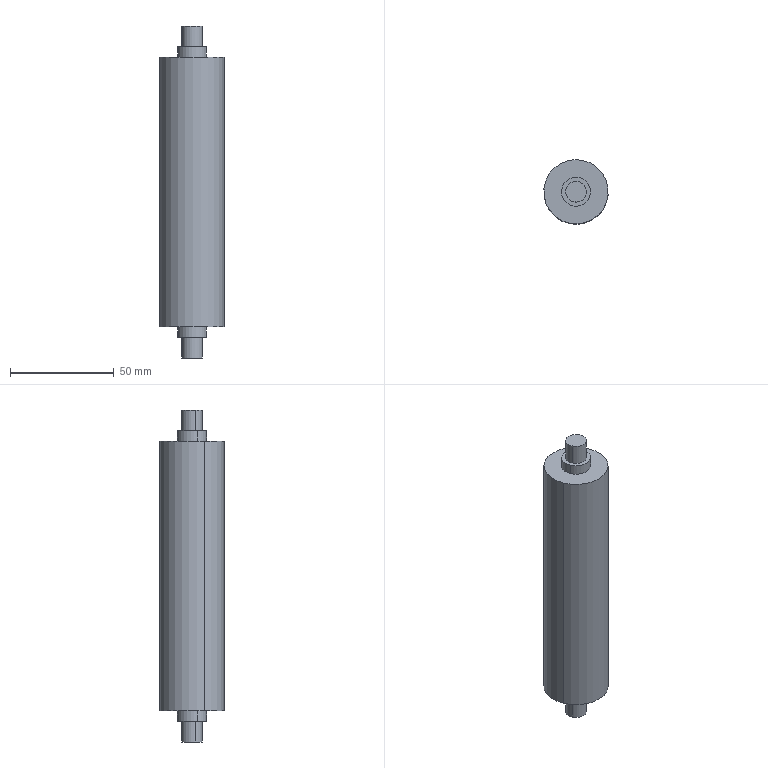Component | SolidWorks | RubberRoller.1-1 | 1 solid | 16 faces | box 31 x 31 x 160 mm | volume 101230 mm3 | cylinder 10 | plane 6 | commonest cylinder face diameters 14 x4 10 x4 31 x2
build123d program:
from build123d import *

# Parameters (mm, degrees)
SKETCH1_2_R         = 16
BOSS_EXTRUDE1_DEPTH = 65
SKETCH2_R           = 7
BOSS_EXTRUDE2_DEPTH = 70
SKETCH4_R           = 5
BOSS_EXTRUDE4_DEPTH = 80
SKETCH1_R           = 17.5
SKETCH1_R_2         = 15.5
CUT_EXTRUDE1_DEPTH  = 70


with BuildPart() as part:
    # Sketch1_2 → Boss-Extrude1 (new, symmetric)
    with BuildSketch(Plane.XY):
        Circle(SKETCH1_2_R)
    extrude(amount=BOSS_EXTRUDE1_DEPTH, both=True)

    # Sketch2 → Boss-Extrude2 (add, symmetric)
    with BuildSketch(Plane.XY):
        Circle(SKETCH2_R)
    extrude(amount=BOSS_EXTRUDE2_DEPTH, both=True)

    # Sketch4 → Boss-Extrude4 (add, symmetric)
    with BuildSketch(Plane.XY):
        Circle(SKETCH4_R)
    extrude(amount=BOSS_EXTRUDE4_DEPTH, both=True)

    # Sketch1 → Cut-Extrude1 (cut, symmetric)
    with BuildSketch(Plane.XY):
        Circle(SKETCH1_R)
        Circle(SKETCH1_R_2, mode=Mode.SUBTRACT)
    extrude(amount=CUT_EXTRUDE1_DEPTH, both=True, mode=Mode.SUBTRACT)


solid = part.part

# Placed as in the assembly
solid = solid.moved(Location((40.5, 166.5, 0), (0, 0, 0)))
STEP:
#1=COLOUR_RGB('',0.7922,0.8196,0.9333);
#2=FILL_AREA_STYLE_COLOUR('',#1);
#3=FILL_AREA_STYLE('',(#2));
#4=SURFACE_STYLE_FILL_AREA(#3);
#5=SURFACE_SIDE_STYLE('',(#4));
#6=SURFACE_STYLE_USAGE(.BOTH.,#5);
#7=PRESENTATION_STYLE_ASSIGNMENT((#6));
#8=CARTESIAN_POINT('',(1.34,6.45,2.559));
#9=VERTEX_POINT('',#8);
#10=CARTESIAN_POINT('',(1.849,6.661,2.559));
#11=VERTEX_POINT('',#10);
#12=CARTESIAN_POINT('',(1.594,6.555,2.559));
#13=DIRECTION('',(0.,0.,1.));
#14=DIRECTION('',(0.9237,0.383,0.));
#15=AXIS2_PLACEMENT_3D('',#12,#13,#14);
#16=CIRCLE('',#15,0.2756);
#17=EDGE_CURVE('',#9,#11,#16,.T.);
#18=ORIENTED_EDGE('',*,*,#17,.T.);
#19=CARTESIAN_POINT('',(1.849,6.661,2.756));
#20=VERTEX_POINT('',#19);
#21=CARTESIAN_POINT('',(1.849,6.661,-2.756));
#22=DIRECTION('',(0.,0.,1.));
#23=VECTOR('',#22,39.37);
#24=LINE('',#21,#23);
#25=EDGE_CURVE('',#11,#20,#24,.T.);
#26=ORIENTED_EDGE('',*,*,#25,.T.);
#27=CARTESIAN_POINT('',(1.34,6.45,2.756));
#28=VERTEX_POINT('',#27);
#29=CARTESIAN_POINT('',(1.594,6.555,2.756));
#30=DIRECTION('',(0.,0.,-1.));
#31=DIRECTION('',(0.9237,0.383,0.));
#32=AXIS2_PLACEMENT_3D('',#29,#30,#31);
#33=CIRCLE('',#32,0.2756);
#34=EDGE_CURVE('',#20,#28,#33,.T.);
#35=ORIENTED_EDGE('',*,*,#34,.T.);
#36=CARTESIAN_POINT('',(1.34,6.45,-2.756));
#37=DIRECTION('',(0.,0.,1.));
#38=VECTOR('',#37,39.37);
#39=LINE('',#36,#38);
#40=EDGE_CURVE('',#9,#28,#39,.T.);
#41=ORIENTED_EDGE('',*,*,#40,.F.);
#42=EDGE_LOOP('',(#18,#26,#35,#41));
#43=FACE_OUTER_BOUND('',#42,.T.);
#44=CARTESIAN_POINT('',(1.594,6.555,-2.756));
#45=DIRECTION('',(0.,0.,1.));
#46=DIRECTION('',(-0.9237,-0.383,0.));
#47=AXIS2_PLACEMENT_3D('',#44,#45,#46);
#48=CYLINDRICAL_SURFACE('',#47,0.2756);
#49=ADVANCED_FACE('',(#43),#48,.T.);
#50=CARTESIAN_POINT('',(1.413,6.48,2.756));
#51=VERTEX_POINT('',#50);
#52=CARTESIAN_POINT('',(1.776,6.631,2.756));
#53=VERTEX_POINT('',#52);
#54=CARTESIAN_POINT('',(1.594,6.555,2.756));
#55=DIRECTION('',(0.,0.,1.));
#56=DIRECTION('',(0.9237,0.383,0.));
#57=AXIS2_PLACEMENT_3D('',#54,#55,#56);
#58=CIRCLE('',#57,0.1969);
#59=EDGE_CURVE('',#51,#53,#58,.T.);
#60=ORIENTED_EDGE('',*,*,#59,.T.);
#61=CARTESIAN_POINT('',(1.776,6.631,3.15));
#62=VERTEX_POINT('',#61);
#63=CARTESIAN_POINT('',(1.776,6.631,-3.15));
#64=DIRECTION('',(0.,0.,1.));
#65=VECTOR('',#64,39.37);
#66=LINE('',#63,#65);
#67=EDGE_CURVE('',#53,#62,#66,.T.);
#68=ORIENTED_EDGE('',*,*,#67,.T.);
#69=CARTESIAN_POINT('',(1.413,6.48,3.15));
#70=VERTEX_POINT('',#69);
#71=CARTESIAN_POINT('',(1.594,6.555,3.15));
#72=DIRECTION('',(0.,0.,-1.));
#73=DIRECTION('',(0.9237,0.383,0.));
#74=AXIS2_PLACEMENT_3D('',#71,#72,#73);
#75=CIRCLE('',#74,0.1969);
#76=EDGE_CURVE('',#62,#70,#75,.T.);
#77=ORIENTED_EDGE('',*,*,#76,.T.);
#78=CARTESIAN_POINT('',(1.413,6.48,-3.15));
#79=DIRECTION('',(0.,0.,1.));
#80=VECTOR('',#79,39.37);
#81=LINE('',#78,#80);
#82=EDGE_CURVE('',#51,#70,#81,.T.);
#83=ORIENTED_EDGE('',*,*,#82,.F.);
#84=EDGE_LOOP('',(#60,#68,#77,#83));
#85=FACE_OUTER_BOUND('',#84,.T.);
#86=CARTESIAN_POINT('',(1.594,6.555,-3.15));
#87=DIRECTION('',(0.,0.,1.));
#88=DIRECTION('',(-0.9237,-0.383,0.));
#89=AXIS2_PLACEMENT_3D('',#86,#87,#88);
#90=CYLINDRICAL_SURFACE('',#89,0.1969);
#91=ADVANCED_FACE('',(#85),#90,.T.);
#92=CARTESIAN_POINT('',(2.158,6.789,2.559));
#93=VERTEX_POINT('',#92);
#94=CARTESIAN_POINT('',(1.031,6.321,2.559));
#95=VERTEX_POINT('',#94);
#96=CARTESIAN_POINT('',(1.594,6.555,2.559));
#97=DIRECTION('',(0.,0.,-1.));
#98=DIRECTION('',(0.9237,0.383,0.));
#99=AXIS2_PLACEMENT_3D('',#96,#97,#98);
#100=CIRCLE('',#99,0.6102);
#101=EDGE_CURVE('',#93,#95,#100,.T.);
#102=ORIENTED_EDGE('',*,*,#101,.T.);
#103=CARTESIAN_POINT('',(1.031,6.321,-2.559));
#104=VERTEX_POINT('',#103);
#105=CARTESIAN_POINT('',(1.031,6.321,2.756));
#106=DIRECTION('',(0.,0.,-1.));
#107=VECTOR('',#106,39.37);
#108=LINE('',#105,#107);
#109=EDGE_CURVE('',#95,#104,#108,.T.);
#110=ORIENTED_EDGE('',*,*,#109,.T.);
#111=CARTESIAN_POINT('',(2.158,6.789,-2.559));
#112=VERTEX_POINT('',#111);
#113=CARTESIAN_POINT('',(1.594,6.555,-2.559));
#114=DIRECTION('',(0.,0.,-1.));
#115=DIRECTION('',(0.9237,0.383,0.));
#116=AXIS2_PLACEMENT_3D('',#113,#114,#115);
#117=CIRCLE('',#116,0.6102);
#118=EDGE_CURVE('',#112,#104,#117,.T.);
#119=ORIENTED_EDGE('',*,*,#118,.F.);
#120=CARTESIAN_POINT('',(2.158,6.789,2.756));
#121=DIRECTION('',(0.,0.,-1.));
#122=VECTOR('',#121,39.37);
#123=LINE('',#120,#122);
#124=EDGE_CURVE('',#93,#112,#123,.T.);
#125=ORIENTED_EDGE('',*,*,#124,.F.);
#126=EDGE_LOOP('',(#102,#110,#119,#125));
#127=FACE_OUTER_BOUND('',#126,.T.);
#128=CARTESIAN_POINT('',(1.594,6.555,2.756));
#129=DIRECTION('',(0.,0.,-1.));
#130=DIRECTION('',(0.9237,0.383,0.));
#131=AXIS2_PLACEMENT_3D('',#128,#129,#130);
#132=CYLINDRICAL_SURFACE('',#131,0.6102);
#133=ADVANCED_FACE('',(#127),#132,.T.);
#134=CARTESIAN_POINT('',(1.776,6.631,-3.15));
#135=VERTEX_POINT('',#134);
#136=CARTESIAN_POINT('',(1.413,6.48,-3.15));
#137=VERTEX_POINT('',#136);
#138=CARTESIAN_POINT('',(1.594,6.555,-3.15));
#139=DIRECTION('',(0.,0.,-1.));
#140=DIRECTION('',(0.9237,0.383,0.));
#141=AXIS2_PLACEMENT_3D('',#138,#139,#140);
#142=CIRCLE('',#141,0.1969);
#143=EDGE_CURVE('',#135,#137,#142,.T.);
#144=ORIENTED_EDGE('',*,*,#143,.F.);
#145=CARTESIAN_POINT('',(1.776,6.631,-2.756));
#146=VERTEX_POINT('',#145);
#147=CARTESIAN_POINT('',(1.776,6.631,-3.15));
#148=DIRECTION('',(0.,0.,1.));
#149=VECTOR('',#148,39.37);
#150=LINE('',#147,#149);
#151=EDGE_CURVE('',#135,#146,#150,.T.);
#152=ORIENTED_EDGE('',*,*,#151,.T.);
#153=CARTESIAN_POINT('',(1.413,6.48,-2.756));
#154=VERTEX_POINT('',#153);
#155=CARTESIAN_POINT('',(1.594,6.555,-2.756));
#156=DIRECTION('',(0.,0.,1.));
#157=DIRECTION('',(0.9237,0.383,0.));
#158=AXIS2_PLACEMENT_3D('',#155,#156,#157);
#159=CIRCLE('',#158,0.1969);
#160=EDGE_CURVE('',#154,#146,#159,.T.);
#161=ORIENTED_EDGE('',*,*,#160,.F.);
#162=CARTESIAN_POINT('',(1.413,6.48,-3.15));
#163=DIRECTION('',(0.,0.,1.));
#164=VECTOR('',#163,39.37);
#165=LINE('',#162,#164);
#166=EDGE_CURVE('',#137,#154,#165,.T.);
#167=ORIENTED_EDGE('',*,*,#166,.F.);
#168=EDGE_LOOP('',(#144,#152,#161,#167));
#169=FACE_OUTER_BOUND('',#168,.T.);
#170=CARTESIAN_POINT('',(1.594,6.555,-3.15));
#171=DIRECTION('',(0.,0.,1.));
#172=DIRECTION('',(-0.9237,-0.383,0.));
#173=AXIS2_PLACEMENT_3D('',#170,#171,#172);
#174=CYLINDRICAL_SURFACE('',#173,0.1969);
#175=ADVANCED_FACE('',(#169),#174,.T.);
#176=CARTESIAN_POINT('',(1.849,6.661,-2.756));
#177=VERTEX_POINT('',#176);
#178=CARTESIAN_POINT('',(1.34,6.45,-2.756));
#179=VERTEX_POINT('',#178);
#180=CARTESIAN_POINT('',(1.594,6.555,-2.756));
#181=DIRECTION('',(0.,0.,-1.));
#182=DIRECTION('',(0.9237,0.383,0.));
#183=AXIS2_PLACEMENT_3D('',#180,#181,#182);
#184=CIRCLE('',#183,0.2756);
#185=EDGE_CURVE('',#177,#179,#184,.T.);
#186=ORIENTED_EDGE('',*,*,#185,.F.);
#187=CARTESIAN_POINT('',(1.849,6.661,-2.559));
#188=VERTEX_POINT('',#187);
#189=CARTESIAN_POINT('',(1.849,6.661,-2.756));
#190=DIRECTION('',(0.,0.,1.));
#191=VECTOR('',#190,39.37);
#192=LINE('',#189,#191);
#193=EDGE_CURVE('',#177,#188,#192,.T.);
#194=ORIENTED_EDGE('',*,*,#193,.T.);
#195=CARTESIAN_POINT('',(1.34,6.45,-2.559));
#196=VERTEX_POINT('',#195);
#197=CARTESIAN_POINT('',(1.594,6.555,-2.559));
#198=DIRECTION('',(0.,0.,1.));
#199=DIRECTION('',(0.9237,0.383,0.));
#200=AXIS2_PLACEMENT_3D('',#197,#198,#199);
#201=CIRCLE('',#200,0.2756);
#202=EDGE_CURVE('',#196,#188,#201,.T.);
#203=ORIENTED_EDGE('',*,*,#202,.F.);
#204=CARTESIAN_POINT('',(1.34,6.45,-2.756));
#205=DIRECTION('',(0.,0.,1.));
#206=VECTOR('',#205,39.37);
#207=LINE('',#204,#206);
#208=EDGE_CURVE('',#179,#196,#207,.T.);
#209=ORIENTED_EDGE('',*,*,#208,.F.);
#210=EDGE_LOOP('',(#186,#194,#203,#209));
#211=FACE_OUTER_BOUND('',#210,.T.);
#212=CARTESIAN_POINT('',(1.594,6.555,-2.756));
#213=DIRECTION('',(0.,0.,1.));
#214=DIRECTION('',(-0.9237,-0.383,0.));
#215=AXIS2_PLACEMENT_3D('',#212,#213,#214);
#216=CYLINDRICAL_SURFACE('',#215,0.2756);
#217=ADVANCED_FACE('',(#211),#216,.T.);
#218=ORIENTED_EDGE('',*,*,#202,.T.);
#219=CARTESIAN_POINT('',(1.594,6.555,-2.559));
#220=DIRECTION('',(0.,0.,1.));
#221=DIRECTION('',(0.9237,0.383,0.));
#222=AXIS2_PLACEMENT_3D('',#219,#220,#221);
#223=CIRCLE('',#222,0.2756);
#224=EDGE_CURVE('',#188,#196,#223,.T.);
#225=ORIENTED_EDGE('',*,*,#224,.T.);
#226=EDGE_LOOP('',(#218,#225));
#227=FACE_BOUND('',#226,.T.);
#228=ORIENTED_EDGE('',*,*,#118,.T.);
#229=CARTESIAN_POINT('',(1.594,6.555,-2.559));
#230=DIRECTION('',(0.,0.,-1.));
#231=DIRECTION('',(0.9237,0.383,0.));
#232=AXIS2_PLACEMENT_3D('',#229,#230,#231);
#233=CIRCLE('',#232,0.6102);
#234=EDGE_CURVE('',#104,#112,#233,.T.);
#235=ORIENTED_EDGE('',*,*,#234,.T.);
#236=EDGE_LOOP('',(#228,#235));
#237=FACE_OUTER_BOUND('',#236,.T.);
#238=CARTESIAN_POINT('',(1.594,6.555,-2.559));
#239=DIRECTION('',(0.,0.,-1.));
#240=DIRECTION('',(0.9237,0.383,0.));
#241=AXIS2_PLACEMENT_3D('',#238,#239,#240);
#242=PLANE('',#241);
#243=ADVANCED_FACE('',(#227,#237),#242,.T.);
#244=CARTESIAN_POINT('',(1.594,6.555,-2.756));
#245=DIRECTION('',(0.,0.,-1.));
#246=DIRECTION('',(0.9237,0.383,0.));
#247=AXIS2_PLACEMENT_3D('',#244,#245,#246);
#248=CIRCLE('',#247,0.2756);
#249=EDGE_CURVE('',#179,#177,#248,.T.);
#250=ORIENTED_EDGE('',*,*,#249,.T.);
#251=ORIENTED_EDGE('',*,*,#185,.T.);
#252=EDGE_LOOP('',(#250,#251));
#253=FACE_OUTER_BOUND('',#252,.T.);
#254=ORIENTED_EDGE('',*,*,#160,.T.);
#255=CARTESIAN_POINT('',(1.594,6.555,-2.756));
#256=DIRECTION('',(0.,0.,1.));
#257=DIRECTION('',(0.9237,0.383,0.));
#258=AXIS2_PLACEMENT_3D('',#255,#256,#257);
#259=CIRCLE('',#258,0.1969);
#260=EDGE_CURVE('',#146,#154,#259,.T.);
#261=ORIENTED_EDGE('',*,*,#260,.T.);
#262=EDGE_LOOP('',(#254,#261));
#263=FACE_BOUND('',#262,.T.);
#264=CARTESIAN_POINT('',(1.594,6.555,-2.756));
#265=DIRECTION('',(0.,0.,-1.));
#266=DIRECTION('',(0.9237,0.383,0.));
#267=AXIS2_PLACEMENT_3D('',#264,#265,#266);
#268=PLANE('',#267);
#269=ADVANCED_FACE('',(#253,#263),#268,.T.);
#270=ORIENTED_EDGE('',*,*,#193,.F.);
#271=ORIENTED_EDGE('',*,*,#249,.F.);
#272=ORIENTED_EDGE('',*,*,#208,.T.);
#273=ORIENTED_EDGE('',*,*,#224,.F.);
#274=EDGE_LOOP('',(#270,#271,#272,#273));
#275=FACE_OUTER_BOUND('',#274,.T.);
#276=CARTESIAN_POINT('',(1.594,6.555,-2.756));
#277=DIRECTION('',(0.,0.,1.));
#278=DIRECTION('',(-0.9237,-0.383,0.));
#279=AXIS2_PLACEMENT_3D('',#276,#277,#278);
#280=CYLINDRICAL_SURFACE('',#279,0.2756);
#281=ADVANCED_FACE('',(#275),#280,.T.);
#282=CARTESIAN_POINT('',(1.594,6.555,-3.15));
#283=DIRECTION('',(0.,0.,-1.));
#284=DIRECTION('',(0.9237,0.383,0.));
#285=AXIS2_PLACEMENT_3D('',#282,#283,#284);
#286=CIRCLE('',#285,0.1969);
#287=EDGE_CURVE('',#137,#135,#286,.T.);
#288=ORIENTED_EDGE('',*,*,#287,.T.);
#289=ORIENTED_EDGE('',*,*,#143,.T.);
#290=EDGE_LOOP('',(#288,#289));
#291=FACE_OUTER_BOUND('',#290,.T.);
#292=CARTESIAN_POINT('',(1.594,6.555,-3.15));
#293=DIRECTION('',(0.,0.,-1.));
#294=DIRECTION('',(0.9237,0.383,0.));
#295=AXIS2_PLACEMENT_3D('',#292,#293,#294);
#296=PLANE('',#295);
#297=ADVANCED_FACE('',(#291),#296,.T.);
#298=ORIENTED_EDGE('',*,*,#151,.F.);
#299=ORIENTED_EDGE('',*,*,#287,.F.);
#300=ORIENTED_EDGE('',*,*,#166,.T.);
#301=ORIENTED_EDGE('',*,*,#260,.F.);
#302=EDGE_LOOP('',(#298,#299,#300,#301));
#303=FACE_OUTER_BOUND('',#302,.T.);
#304=CARTESIAN_POINT('',(1.594,6.555,-3.15));
#305=DIRECTION('',(0.,0.,1.));
#306=DIRECTION('',(-0.9237,-0.383,0.));
#307=AXIS2_PLACEMENT_3D('',#304,#305,#306);
#308=CYLINDRICAL_SURFACE('',#307,0.1969);
#309=ADVANCED_FACE('',(#303),#308,.T.);
#310=ORIENTED_EDGE('',*,*,#109,.F.);
#311=CARTESIAN_POINT('',(1.594,6.555,2.559));
#312=DIRECTION('',(0.,0.,-1.));
#313=DIRECTION('',(0.9237,0.383,0.));
#314=AXIS2_PLACEMENT_3D('',#311,#312,#313);
#315=CIRCLE('',#314,0.6102);
#316=EDGE_CURVE('',#95,#93,#315,.T.);
#317=ORIENTED_EDGE('',*,*,#316,.T.);
#318=ORIENTED_EDGE('',*,*,#124,.T.);
#319=ORIENTED_EDGE('',*,*,#234,.F.);
#320=EDGE_LOOP('',(#310,#317,#318,#319));
#321=FACE_OUTER_BOUND('',#320,.T.);
#322=CARTESIAN_POINT('',(1.594,6.555,2.756));
#323=DIRECTION('',(0.,0.,-1.));
#324=DIRECTION('',(0.9237,0.383,0.));
#325=AXIS2_PLACEMENT_3D('',#322,#323,#324);
#326=CYLINDRICAL_SURFACE('',#325,0.6102);
#327=ADVANCED_FACE('',(#321),#326,.T.);
#328=CARTESIAN_POINT('',(1.594,6.555,3.15));
#329=DIRECTION('',(0.,0.,-1.));
#330=DIRECTION('',(0.9237,0.383,0.));
#331=AXIS2_PLACEMENT_3D('',#328,#329,#330);
#332=CIRCLE('',#331,0.1969);
#333=EDGE_CURVE('',#70,#62,#332,.T.);
#334=ORIENTED_EDGE('',*,*,#333,.F.);
#335=ORIENTED_EDGE('',*,*,#76,.F.);
#336=EDGE_LOOP('',(#334,#335));
#337=FACE_OUTER_BOUND('',#336,.T.);
#338=CARTESIAN_POINT('',(1.594,6.555,3.15));
#339=DIRECTION('',(0.,0.,-1.));
#340=DIRECTION('',(0.9237,0.383,0.));
#341=AXIS2_PLACEMENT_3D('',#338,#339,#340);
#342=PLANE('',#341);
#343=ADVANCED_FACE('',(#337),#342,.F.);
#344=ORIENTED_EDGE('',*,*,#67,.F.);
#345=CARTESIAN_POINT('',(1.594,6.555,2.756));
#346=DIRECTION('',(0.,0.,1.));
#347=DIRECTION('',(0.9237,0.383,0.));
#348=AXIS2_PLACEMENT_3D('',#345,#346,#347);
#349=CIRCLE('',#348,0.1969);
#350=EDGE_CURVE('',#53,#51,#349,.T.);
#351=ORIENTED_EDGE('',*,*,#350,.T.);
#352=ORIENTED_EDGE('',*,*,#82,.T.);
#353=ORIENTED_EDGE('',*,*,#333,.T.);
#354=EDGE_LOOP('',(#344,#351,#352,#353));
#355=FACE_OUTER_BOUND('',#354,.T.);
#356=CARTESIAN_POINT('',(1.594,6.555,-3.15));
#357=DIRECTION('',(0.,0.,1.));
#358=DIRECTION('',(-0.9237,-0.383,0.));
#359=AXIS2_PLACEMENT_3D('',#356,#357,#358);
#360=CYLINDRICAL_SURFACE('',#359,0.1969);
#361=ADVANCED_FACE('',(#355),#360,.T.);
#362=CARTESIAN_POINT('',(1.594,6.555,2.756));
#363=DIRECTION('',(0.,0.,-1.));
#364=DIRECTION('',(0.9237,0.383,0.));
#365=AXIS2_PLACEMENT_3D('',#362,#363,#364);
#366=CIRCLE('',#365,0.2756);
#367=EDGE_CURVE('',#28,#20,#366,.T.);
#368=ORIENTED_EDGE('',*,*,#367,.F.);
#369=ORIENTED_EDGE('',*,*,#34,.F.);
#370=EDGE_LOOP('',(#368,#369));
#371=FACE_OUTER_BOUND('',#370,.T.);
#372=ORIENTED_EDGE('',*,*,#59,.F.);
#373=ORIENTED_EDGE('',*,*,#350,.F.);
#374=EDGE_LOOP('',(#372,#373));
#375=FACE_BOUND('',#374,.T.);
#376=CARTESIAN_POINT('',(1.594,6.555,2.756));
#377=DIRECTION('',(0.,0.,-1.));
#378=DIRECTION('',(0.9237,0.383,0.));
#379=AXIS2_PLACEMENT_3D('',#376,#377,#378);
#380=PLANE('',#379);
#381=ADVANCED_FACE('',(#371,#375),#380,.F.);
#382=ORIENTED_EDGE('',*,*,#25,.F.);
#383=CARTESIAN_POINT('',(1.594,6.555,2.559));
#384=DIRECTION('',(0.,0.,1.));
#385=DIRECTION('',(0.9237,0.383,0.));
#386=AXIS2_PLACEMENT_3D('',#383,#384,#385);
#387=CIRCLE('',#386,0.2756);
#388=EDGE_CURVE('',#11,#9,#387,.T.);
#389=ORIENTED_EDGE('',*,*,#388,.T.);
#390=ORIENTED_EDGE('',*,*,#40,.T.);
#391=ORIENTED_EDGE('',*,*,#367,.T.);
#392=EDGE_LOOP('',(#382,#389,#390,#391));
#393=FACE_OUTER_BOUND('',#392,.T.);
#394=CARTESIAN_POINT('',(1.594,6.555,-2.756));
#395=DIRECTION('',(0.,0.,1.));
#396=DIRECTION('',(-0.9237,-0.383,0.));
#397=AXIS2_PLACEMENT_3D('',#394,#395,#396);
#398=CYLINDRICAL_SURFACE('',#397,0.2756);
#399=ADVANCED_FACE('',(#393),#398,.T.);
#400=ORIENTED_EDGE('',*,*,#17,.F.);
#401=ORIENTED_EDGE('',*,*,#388,.F.);
#402=EDGE_LOOP('',(#400,#401));
#403=FACE_BOUND('',#402,.T.);
#404=ORIENTED_EDGE('',*,*,#101,.F.);
#405=ORIENTED_EDGE('',*,*,#316,.F.);
#406=EDGE_LOOP('',(#404,#405));
#407=FACE_OUTER_BOUND('',#406,.T.);
#408=CARTESIAN_POINT('',(1.594,6.555,2.559));
#409=DIRECTION('',(0.,0.,-1.));
#410=DIRECTION('',(0.9237,0.383,0.));
#411=AXIS2_PLACEMENT_3D('',#408,#409,#410);
#412=PLANE('',#411);
#413=ADVANCED_FACE('',(#403,#407),#412,.F.);
#414=CLOSED_SHELL('',(#49,#91,#133,#175,#217,#243,#269,#281,#297,#309,#327,#343,#361,#381,#399,#413));
#415=MANIFOLD_SOLID_BREP('',#414);
#416=STYLED_ITEM('',(#7),#415);
#417=PRESENTATION_LAYER_ASSIGNMENT('','',(#416));
#418=(LENGTH_UNIT()NAMED_UNIT(*)SI_UNIT($,.METRE.));
#419=LENGTH_MEASURE_WITH_UNIT(LENGTH_MEASURE(0.0254),#418);
#420=DIMENSIONAL_EXPONENTS(1.,0.,0.,0.,0.,0.,0.);
#421=(CONVERSION_BASED_UNIT('',#419)LENGTH_UNIT()NAMED_UNIT(#420));
#422=UNCERTAINTY_MEASURE_WITH_UNIT(LENGTH_MEASURE(0.00001),#421,'','');
#423=(NAMED_UNIT(*)PLANE_ANGLE_UNIT()SI_UNIT($,.RADIAN.));
#424=(NAMED_UNIT(*)SI_UNIT($,.STERADIAN.)SOLID_ANGLE_UNIT());
#425=(GEOMETRIC_REPRESENTATION_CONTEXT(3)GLOBAL_UNCERTAINTY_ASSIGNED_CONTEXT((#422))GLOBAL_UNIT_ASSIGNED_CONTEXT((#421,#423,#424))REPRESENTATION_CONTEXT('',''));
#426=MECHANICAL_DESIGN_GEOMETRIC_PRESENTATION_REPRESENTATION('',(#416),#425);
#427=CARTESIAN_POINT('',(0.,0.,0.));
#428=DIRECTION('',(0.,0.,1.));
#429=DIRECTION('',(1.,0.,0.));
#430=AXIS2_PLACEMENT_3D('',#427,#428,#429);
#431=(LENGTH_UNIT()NAMED_UNIT(*)SI_UNIT($,.METRE.));
#432=LENGTH_MEASURE_WITH_UNIT(LENGTH_MEASURE(0.0254),#431);
#433=DIMENSIONAL_EXPONENTS(1.,0.,0.,0.,0.,0.,0.);
#434=(CONVERSION_BASED_UNIT('',#432)LENGTH_UNIT()NAMED_UNIT(#433));
#435=UNCERTAINTY_MEASURE_WITH_UNIT(LENGTH_MEASURE(0.00001),#434,'','');
#436=(NAMED_UNIT(*)PLANE_ANGLE_UNIT()SI_UNIT($,.RADIAN.));
#437=(NAMED_UNIT(*)SI_UNIT($,.STERADIAN.)SOLID_ANGLE_UNIT());
#438=(GEOMETRIC_REPRESENTATION_CONTEXT(3)GLOBAL_UNCERTAINTY_ASSIGNED_CONTEXT((#435))GLOBAL_UNIT_ASSIGNED_CONTEXT((#434,#436,#437))REPRESENTATION_CONTEXT('',''));
#439=ADVANCED_BREP_SHAPE_REPRESENTATION('',(#415,#430),#438);